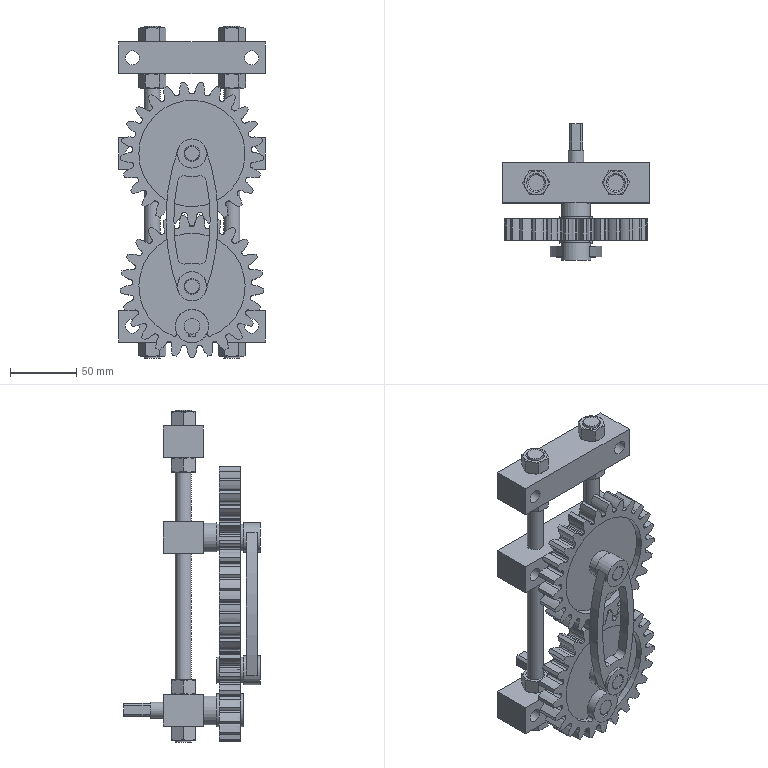Assembly | NX | mm | 19 component files | 20 solids | 612 faces | box 110 x 103 x 250 mm | volume 469556 mm3 | plane 132 | other 125 | spline 125 | cone 116 | cylinder 114 | commonest cylinder face diameters 12 x26 90 x25 89.84 x25 10.5 x6 22 x4 5 x4 80 x4 20 x4
Bill of materials:
unnamed part 1 | 1 |  | Elongated, flat, lens-shaped link plate with a large central oblong opening and a round through hole at each rounded end.
unnamed part 2 | 2 |  | Long, slender, plain solid cylindrical rod with flat ends.
unnamed part 3 | 1 |  | Spur-type toothed gear disc with straight teeth, a central round bore, and a second off-center bore that has a keyway-like notch. Both bores are surrounded by raised hub bosses.
unnamed part 4 | 2 |  | Rectangular bar block with two vertical through holes, two horizontal cross holes near the ends, and a hollow cylindrical boss sticking out from the middle of one long side face.
GB-T6170_F-2000,M12x1.75 | 8 |  | Hexagonal nut-shaped body with a large central round bore and chamfered corners on both faces.
GB-T119.1-2000,12x70 | 1 |  | Parallel Pin, GB-T 119.1-2000,12x70
unnamed part 5 | 1 |  | Plain rectangular bar block with two vertical through holes and two horizontal cross holes near the ends.
unnamed part 6 | 1 |  | Stepped cylindrical shaft with a reduced-diameter section at one end and a small radial projection near the opposite end.
unnamed part 7 | 1 |  | Spur-type toothed gear disc with straight teeth, a single central round bore, and a small cylindrical hub boss.
GB-T119.1-2000,12x32 | 1 |  | Parallel Pin, GB-T 119.1-2000,12x32
Mates:
1. fix | smooth_shaft 2 component
2. touch align | support_block 1 face | smooth_shaft 2 face
3. distance | support_block 1 face | smooth_shaft 2 face
4. touch align | moving_block 2 face | smooth_shaft 2 face
5. distance | moving_block 2 face | smooth_shaft 2 face
6. bond | support_block 1 component | assembly component
7. bond | smooth_shaft 2 component | assembly component
8. bond | smooth_shaft 1 component | assembly component
9. linear | assembly datumaxis | assembly cartesiancoordinatesystem | assembly cartesiancoordinatesystem
10. concentric | connecting_rod 1 edge | guide_gear 1 edge
11. concentric | connecting_rod 1 edge | eccentric_gear 1 edge
12. concentric | eccentric_gear 1 edge | moving_block 2 edge
13. fix | eccentric_gear 1 component
14. concentric | moving_block 1 edge | guide_gear 1 edge
15. touch align | moving_block 1 face | smooth_shaft 2 face
16. concentric | shaft 1 edge | eccentric_gear 1 edge
17. concentric | GB-T6170_F-2000_M12x1_75 3 edge | support_block 1 edge
18. concentric | GB-T6170_F-2000_M12x1_75 4 edge | support_block 1 edge
19. concentric | GB-T6170_F-2000_M12x1_75 6 edge | moving_block 2 edge
20. concentric | GB-T6170_F-2000_M12x1_75 5 edge | moving_block 2 edge
21. concentric | GB-T6170_F-2000_M12x1_75 7 edge | moving_block 2 edge
22. concentric | GB-T6170_F-2000_M12x1_75 8 edge | moving_block 2 edge
23. concentric | GB-T6170_F-2000_M12x1_75 1 edge | support_block 1 edge
24. concentric | support_block 1 edge | GB-T6170_F-2000_M12x1_75 2 edge